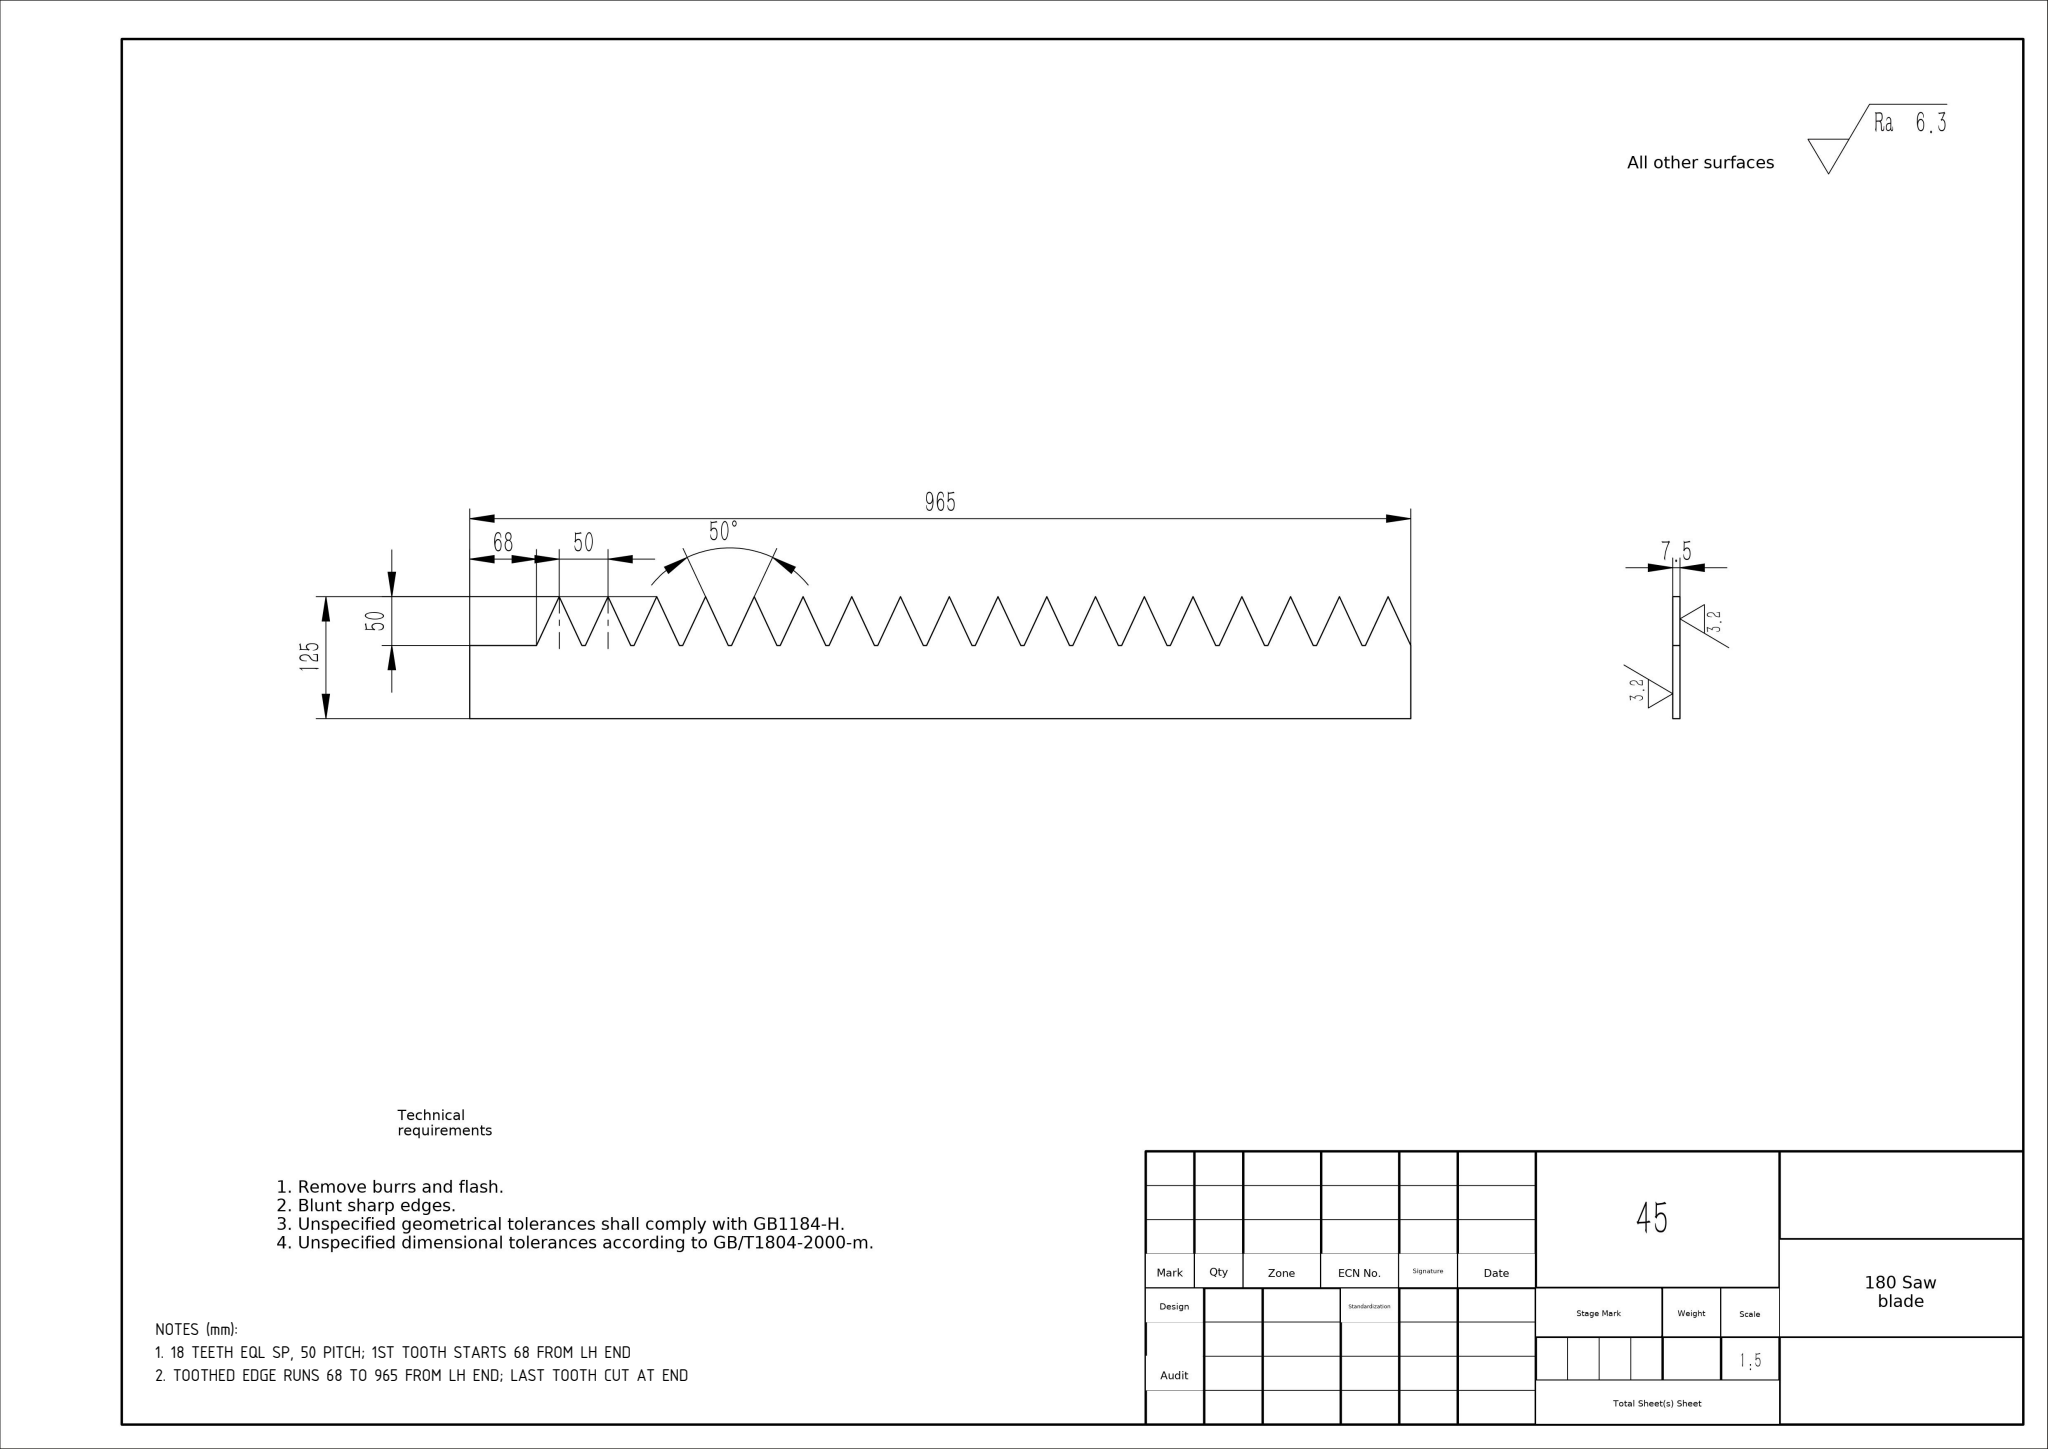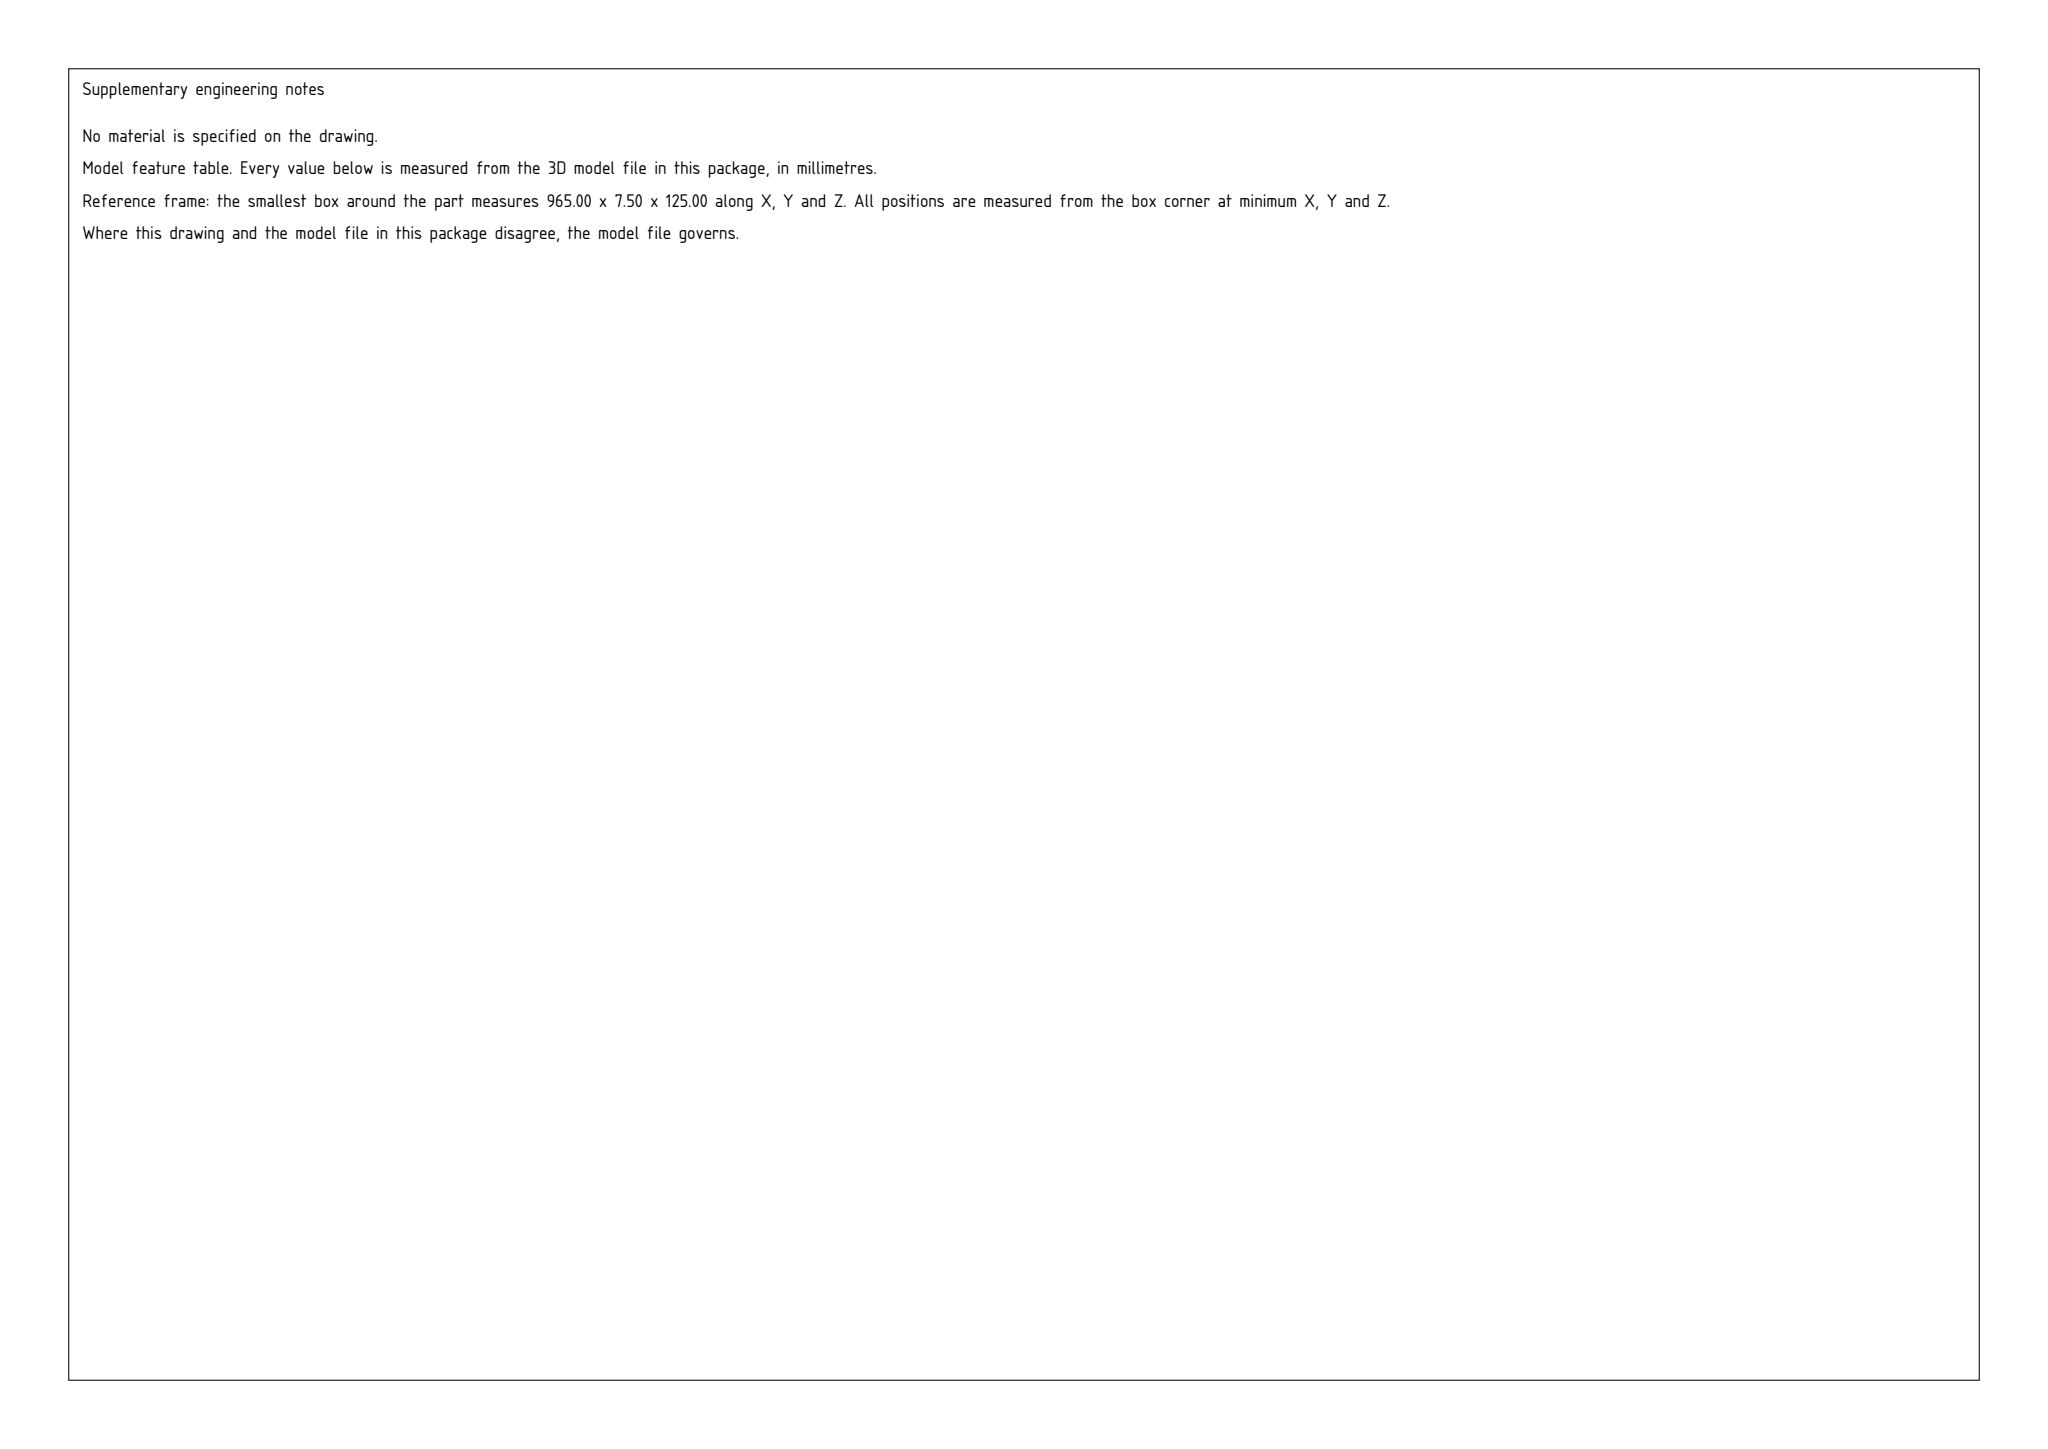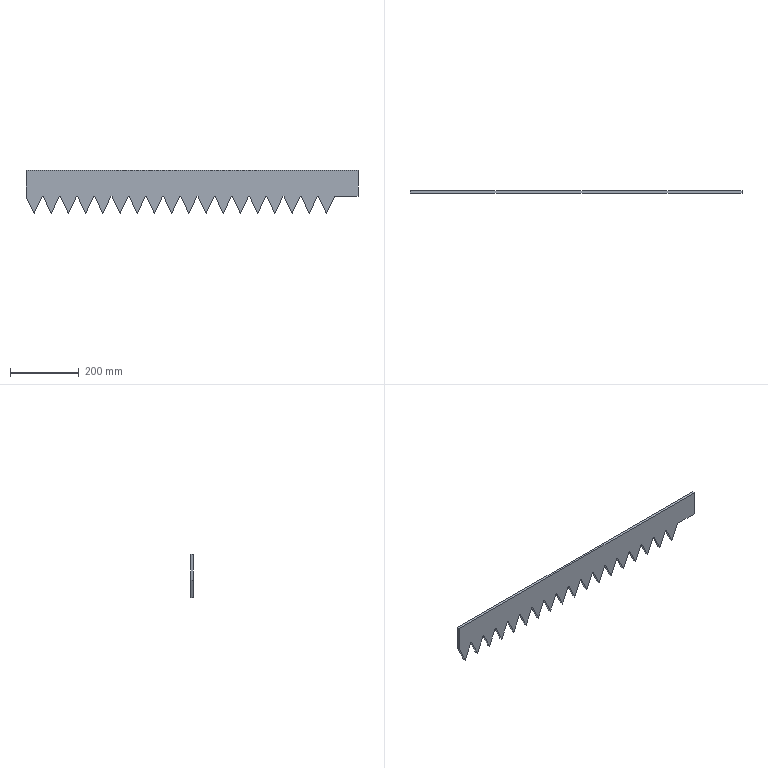Part | SolidWorks | mm | 1 solid | 59 faces | box 965 x 7.5 x 125 mm | volume 700191 mm3 | plane 59
Drawing notes:
18 TEETH EQL SP, 50 PITCH; 1ST TOOTH STARTS 68 FROM LH END | from the solid: 18 planar faces at z=50 (gullet/land level, 50 below tooth tips); pitch 50 from x=68 gives 18 teeth within 965 length
TOOTHED EDGE RUNS 68 TO 965 FROM LH END; LAST TOOTH CUT AT END | from the solid: bbox_xyz x=965, planes x=0 and x=965; teeth start 68 from x=0; (965-68)/50 = 17.94 so final tooth truncated by end face
build123d program:
from build123d import *

# Parameters (mm, degrees)
SKETCH1_W           = 193
SKETCH1_H           = 15
BOSS_EXTRUDE1_DEPTH = 1.5
BOSS_EXTRUDE2_DEPTH = 1.5
SCALE1_SCALE        = 5


with BuildPart() as part:
    # Sketch1 → Boss-Extrude1 (new body)
    with BuildSketch(Plane(origin=(0, 0, 0), x_dir=(1, 0, 0), z_dir=(0, 1, 0))):
        with Locations((96.5, -7.5)):
            Rectangle(SKETCH1_W, SKETCH1_H)
    extrude(amount=BOSS_EXTRUDE1_DEPTH)

    # Sketch2 → Boss-Extrude2 (add)
    with BuildSketch(Plane(origin=(0, 1.5, 0), x_dir=(1, 0, 0), z_dir=(0, 1, 0))):
        Polygon((0, 0), (4.663, 10), (9.326, 0), align=None)
        Polygon((14.663, 10), (19.326, 0), (10, 0), align=None)
        Polygon((24.663, 10), (29.326, 0), (20, 0), align=None)
        Polygon((34.663, 10), (39.326, 0), (30, 0), align=None)
        Polygon((44.663, 10), (49.326, 0), (40, 0), align=None)
        Polygon((54.663, 10), (59.326, 0), (50, 0), align=None)
        Polygon((64.663, 10), (69.326, 0), (60, 0), align=None)
        Polygon((74.663, 10), (79.326, 0), (70, 0), align=None)
        Polygon((84.663, 10), (89.326, 0), (80, 0), align=None)
        Polygon((94.663, 10), (99.326, 0), (90, 0), align=None)
        Polygon((104.663, 10), (109.326, 0), (100, 0), align=None)
        Polygon((114.663, 10), (119.326, 0), (110, 0), align=None)
        Polygon((124.663, 10), (129.326, 0), (120, 0), align=None)
        Polygon((134.663, 10), (139.326, 0), (130, 0), align=None)
        Polygon((144.663, 10), (149.326, 0), (140, 0), align=None)
        Polygon((154.663, 10), (159.326, 0), (150, 0), align=None)
        Polygon((164.663, 10), (169.326, 0), (160, 0), align=None)
        Polygon((174.663, 10), (179.326, 0), (170, 0), align=None)
    extrude(amount=-BOSS_EXTRUDE2_DEPTH)


with BuildPart() as part_1:
    # Scale1: scaled about (94.963, 0.75, 5.065)
    add(part.part.scale(SCALE1_SCALE).moved(Location((-379.853, -3, -20.26))))


solid = part_1.part